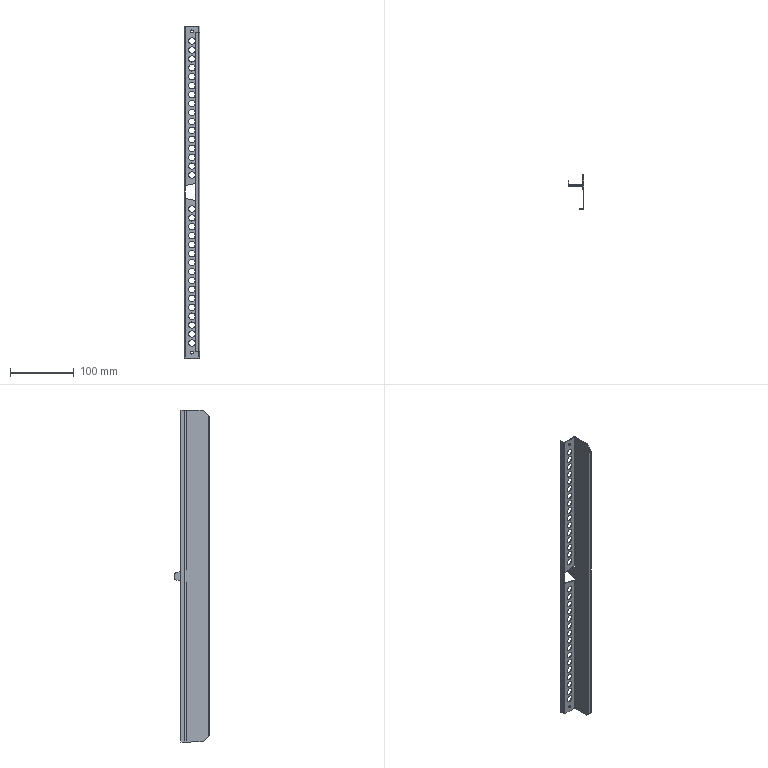Component | SolidWorks | RAY MONTAJ-1_tepsi _st kademeli-1 | 1 solid | 122 faces | volume 34609 mm3 | cylinder 78 | plane 44 | commonest cylinder face diameters 10 x64 4.5 x4 3.473 x4 1.473 x4 6 x2